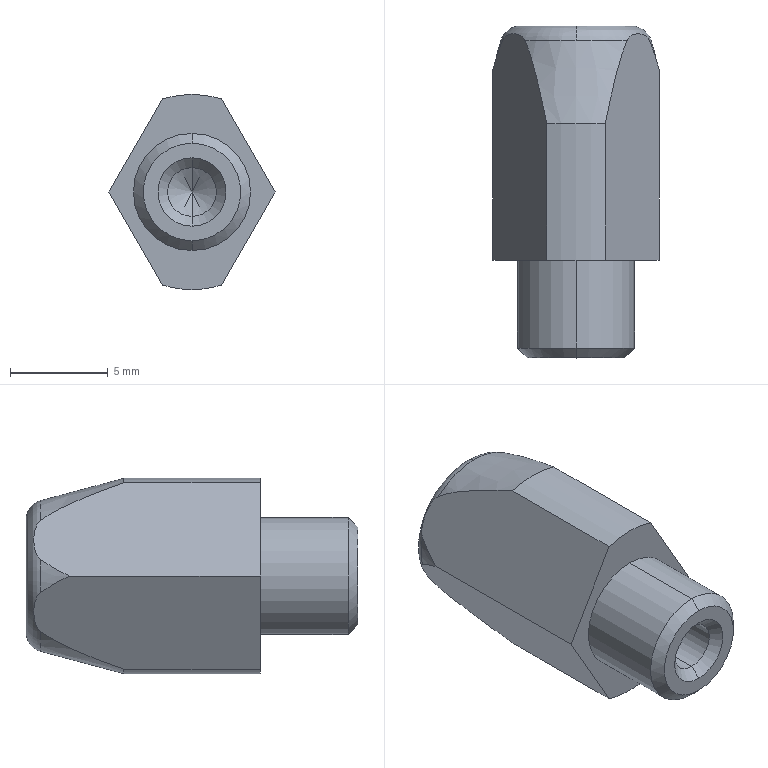Component | SolidWorks | MA060.03.03-05-2 | 1 solid | 27 faces | box 8.51 x 17 x 10 mm | volume 740 mm3 | cone 11 | cylinder 7 | plane 7 | torus 2 | commonest cylinder face diameters 10 x3 2.5 x2 6 x2 | material 45#
STEP:
#1=COLOUR_RGB('',0.7922,0.8196,0.9333);
#2=FILL_AREA_STYLE_COLOUR('',#1);
#3=FILL_AREA_STYLE('',(#2));
#4=SURFACE_STYLE_FILL_AREA(#3);
#5=SURFACE_SIDE_STYLE('',(#4));
#6=SURFACE_STYLE_USAGE(.BOTH.,#5);
#7=PRESENTATION_STYLE_ASSIGNMENT((#6));
#8=CARTESIAN_POINT('',(1.614,3.516,-0.1519));
#9=VERTEX_POINT('',#8);
#10=CARTESIAN_POINT('',(1.717,3.516,-0.1117));
#11=VERTEX_POINT('',#10);
#12=CARTESIAN_POINT('',(1.614,3.516,-0.));
#13=DIRECTION('',(0.,-1.,0.));
#14=DIRECTION('',(0.,0.,1.));
#15=AXIS2_PLACEMENT_3D('',#12,#13,#14);
#16=CIRCLE('',#15,0.1519);
#17=EDGE_CURVE('',#9,#11,#16,.T.);
#18=ORIENTED_EDGE('',*,*,#17,.F.);
#19=CARTESIAN_POINT('',(1.614,3.545,-0.1139));
#20=VERTEX_POINT('',#19);
#21=CARTESIAN_POINT('',(1.614,3.506,-0.1139));
#22=DIRECTION('',(1.,0.,0.));
#23=DIRECTION('',(0.,0.,-1.));
#24=AXIS2_PLACEMENT_3D('',#21,#22,#23);
#25=CIRCLE('',#24,0.03937);
#26=EDGE_CURVE('',#9,#20,#25,.T.);
#27=ORIENTED_EDGE('',*,*,#26,.T.);
#28=CARTESIAN_POINT('',(1.614,3.545,0.1139));
#29=VERTEX_POINT('',#28);
#30=CARTESIAN_POINT('',(1.614,3.545,-0.));
#31=DIRECTION('',(0.,1.,0.));
#32=DIRECTION('',(0.,0.,1.));
#33=AXIS2_PLACEMENT_3D('',#30,#31,#32);
#34=CIRCLE('',#33,0.1139);
#35=EDGE_CURVE('',#29,#20,#34,.T.);
#36=ORIENTED_EDGE('',*,*,#35,.F.);
#37=CARTESIAN_POINT('',(1.614,3.516,0.1519));
#38=VERTEX_POINT('',#37);
#39=CARTESIAN_POINT('',(1.614,3.506,0.1139));
#40=DIRECTION('',(-1.,0.,0.));
#41=DIRECTION('',(0.,0.,1.));
#42=AXIS2_PLACEMENT_3D('',#39,#40,#41);
#43=CIRCLE('',#42,0.03937);
#44=EDGE_CURVE('',#38,#29,#43,.T.);
#45=ORIENTED_EDGE('',*,*,#44,.F.);
#46=CARTESIAN_POINT('',(1.717,3.516,0.1117));
#47=VERTEX_POINT('',#46);
#48=CARTESIAN_POINT('',(1.614,3.516,-0.));
#49=DIRECTION('',(0.,-1.,0.));
#50=DIRECTION('',(0.,0.,1.));
#51=AXIS2_PLACEMENT_3D('',#48,#49,#50);
#52=CIRCLE('',#51,0.1519);
#53=EDGE_CURVE('',#47,#38,#52,.T.);
#54=ORIENTED_EDGE('',*,*,#53,.F.);
#55=CARTESIAN_POINT('',(1.762,3.516,0.03335));
#56=VERTEX_POINT('',#55);
#57=CARTESIAN_POINT('',(1.762,3.516,0.03335));
#58=CARTESIAN_POINT('',(1.761,3.519,0.03573));
#59=CARTESIAN_POINT('',(1.759,3.521,0.0387));
#60=CARTESIAN_POINT('',(1.756,3.525,0.04504));
#61=CARTESIAN_POINT('',(1.754,3.526,0.04835));
#62=CARTESIAN_POINT('',(1.748,3.529,0.05852));
#63=CARTESIAN_POINT('',(1.744,3.53,0.06554));
#64=CARTESIAN_POINT('',(1.736,3.53,0.07943));
#65=CARTESIAN_POINT('',(1.732,3.529,0.08647));
#66=CARTESIAN_POINT('',(1.726,3.526,0.09665));
#67=CARTESIAN_POINT('',(1.724,3.525,0.1));
#68=CARTESIAN_POINT('',(1.72,3.521,0.1063));
#69=CARTESIAN_POINT('',(1.719,3.519,0.1093));
#70=CARTESIAN_POINT('',(1.717,3.516,0.1117));
#71=B_SPLINE_CURVE_WITH_KNOTS('',3,(#57,#58,#59,#60,#61,#62,#63,#64,#65,#66,#67,#68,#69,#70),.UNSPECIFIED.,.F.,.F.,(4,2,2,2,2,2,4),(0.,0.0003075,0.0006151,0.00123,0.001845,0.002153,0.00246),.UNSPECIFIED.);
#72=EDGE_CURVE('',#56,#47,#71,.T.);
#73=ORIENTED_EDGE('',*,*,#72,.F.);
#74=CARTESIAN_POINT('',(1.762,3.516,-0.03335));
#75=VERTEX_POINT('',#74);
#76=CARTESIAN_POINT('',(1.614,3.516,-0.));
#77=DIRECTION('',(0.,-1.,0.));
#78=DIRECTION('',(0.,0.,1.));
#79=AXIS2_PLACEMENT_3D('',#76,#77,#78);
#80=CIRCLE('',#79,0.1519);
#81=EDGE_CURVE('',#75,#56,#80,.T.);
#82=ORIENTED_EDGE('',*,*,#81,.F.);
#83=CARTESIAN_POINT('',(1.717,3.516,-0.1117));
#84=CARTESIAN_POINT('',(1.719,3.519,-0.1093));
#85=CARTESIAN_POINT('',(1.72,3.521,-0.1063));
#86=CARTESIAN_POINT('',(1.724,3.525,-0.1));
#87=CARTESIAN_POINT('',(1.726,3.526,-0.09669));
#88=CARTESIAN_POINT('',(1.732,3.529,-0.08651));
#89=CARTESIAN_POINT('',(1.736,3.53,-0.07949));
#90=CARTESIAN_POINT('',(1.744,3.53,-0.06561));
#91=CARTESIAN_POINT('',(1.748,3.529,-0.05856));
#92=CARTESIAN_POINT('',(1.754,3.526,-0.04838));
#93=CARTESIAN_POINT('',(1.756,3.525,-0.04502));
#94=CARTESIAN_POINT('',(1.759,3.521,-0.03873));
#95=CARTESIAN_POINT('',(1.761,3.519,-0.03572));
#96=CARTESIAN_POINT('',(1.762,3.516,-0.03335));
#97=B_SPLINE_CURVE_WITH_KNOTS('',3,(#83,#84,#85,#86,#87,#88,#89,#90,#91,#92,#93,#94,#95,#96),.UNSPECIFIED.,.F.,.F.,(4,2,2,2,2,2,4),(0.,0.0003075,0.0006151,0.00123,0.001845,0.002153,0.00246),.UNSPECIFIED.);
#98=EDGE_CURVE('',#11,#75,#97,.T.);
#99=ORIENTED_EDGE('',*,*,#98,.F.);
#100=EDGE_LOOP('',(#18,#27,#36,#45,#54,#73,#82,#99));
#101=FACE_OUTER_BOUND('',#100,.T.);
#102=CARTESIAN_POINT('',(1.614,3.506,-0.));
#103=DIRECTION('',(0.,1.,0.));
#104=DIRECTION('',(0.,0.,1.));
#105=AXIS2_PLACEMENT_3D('',#102,#103,#104);
#106=TOROIDAL_SURFACE('',#105,0.1139,0.03937);
#107=ADVANCED_FACE('',(#101),#106,.T.);
#108=CARTESIAN_POINT('',(1.614,2.896,0.04921));
#109=VERTEX_POINT('',#108);
#110=CARTESIAN_POINT('',(1.614,2.896,-0.04921));
#111=VERTEX_POINT('',#110);
#112=CARTESIAN_POINT('',(1.614,2.896,-0.));
#113=DIRECTION('',(0.,-1.,0.));
#114=DIRECTION('',(0.,0.,-1.));
#115=AXIS2_PLACEMENT_3D('',#112,#113,#114);
#116=CIRCLE('',#115,0.04921);
#117=EDGE_CURVE('',#109,#111,#116,.T.);
#118=ORIENTED_EDGE('',*,*,#117,.F.);
#119=CARTESIAN_POINT('',(1.614,2.876,0.0689));
#120=VERTEX_POINT('',#119);
#121=CARTESIAN_POINT('',(1.614,2.896,0.04921));
#122=DIRECTION('',(0.,-0.7071,0.7071));
#123=VECTOR('',#122,39.37);
#124=LINE('',#121,#123);
#125=EDGE_CURVE('',#109,#120,#124,.T.);
#126=ORIENTED_EDGE('',*,*,#125,.T.);
#127=CARTESIAN_POINT('',(1.614,2.876,-0.0689));
#128=VERTEX_POINT('',#127);
#129=CARTESIAN_POINT('',(1.614,2.876,-0.));
#130=DIRECTION('',(0.,1.,0.));
#131=DIRECTION('',(0.,0.,-1.));
#132=AXIS2_PLACEMENT_3D('',#129,#130,#131);
#133=CIRCLE('',#132,0.0689);
#134=EDGE_CURVE('',#128,#120,#133,.T.);
#135=ORIENTED_EDGE('',*,*,#134,.F.);
#136=CARTESIAN_POINT('',(1.614,2.896,-0.04921));
#137=DIRECTION('',(0.,-0.7071,-0.7071));
#138=VECTOR('',#137,39.37);
#139=LINE('',#136,#138);
#140=EDGE_CURVE('',#111,#128,#139,.T.);
#141=ORIENTED_EDGE('',*,*,#140,.F.);
#142=EDGE_LOOP('',(#118,#126,#135,#141));
#143=FACE_OUTER_BOUND('',#142,.T.);
#144=CARTESIAN_POINT('',(1.614,2.896,-0.));
#145=DIRECTION('',(0.,-1.,0.));
#146=DIRECTION('',(0.,0.,-1.));
#147=AXIS2_PLACEMENT_3D('',#144,#145,#146);
#148=CONICAL_SURFACE('',#147,0.04921,0.7854);
#149=ADVANCED_FACE('',(#143),#148,.F.);
#150=CARTESIAN_POINT('',(1.614,2.876,-0.09843));
#151=VERTEX_POINT('',#150);
#152=CARTESIAN_POINT('',(1.614,2.876,0.09843));
#153=VERTEX_POINT('',#152);
#154=CARTESIAN_POINT('',(1.614,2.876,-0.));
#155=DIRECTION('',(0.,-1.,0.));
#156=DIRECTION('',(0.,0.,-1.));
#157=AXIS2_PLACEMENT_3D('',#154,#155,#156);
#158=CIRCLE('',#157,0.09843);
#159=EDGE_CURVE('',#151,#153,#158,.T.);
#160=ORIENTED_EDGE('',*,*,#159,.F.);
#161=CARTESIAN_POINT('',(1.614,2.896,-0.1181));
#162=VERTEX_POINT('',#161);
#163=CARTESIAN_POINT('',(1.614,2.876,-0.09843));
#164=DIRECTION('',(0.,0.7071,-0.7071));
#165=VECTOR('',#164,39.37);
#166=LINE('',#163,#165);
#167=EDGE_CURVE('',#151,#162,#166,.T.);
#168=ORIENTED_EDGE('',*,*,#167,.T.);
#169=CARTESIAN_POINT('',(1.614,2.896,0.1181));
#170=VERTEX_POINT('',#169);
#171=CARTESIAN_POINT('',(1.614,2.896,-0.));
#172=DIRECTION('',(0.,1.,0.));
#173=DIRECTION('',(0.,0.,-1.));
#174=AXIS2_PLACEMENT_3D('',#171,#172,#173);
#175=CIRCLE('',#174,0.1181);
#176=EDGE_CURVE('',#170,#162,#175,.T.);
#177=ORIENTED_EDGE('',*,*,#176,.F.);
#178=CARTESIAN_POINT('',(1.614,2.876,0.09843));
#179=DIRECTION('',(0.,0.7071,0.7071));
#180=VECTOR('',#179,39.37);
#181=LINE('',#178,#180);
#182=EDGE_CURVE('',#153,#170,#181,.T.);
#183=ORIENTED_EDGE('',*,*,#182,.F.);
#184=EDGE_LOOP('',(#160,#168,#177,#183));
#185=FACE_OUTER_BOUND('',#184,.T.);
#186=CARTESIAN_POINT('',(1.614,2.876,-0.));
#187=DIRECTION('',(0.,1.,0.));
#188=DIRECTION('',(0.,0.,1.));
#189=AXIS2_PLACEMENT_3D('',#186,#187,#188);
#190=CONICAL_SURFACE('',#189,0.09843,0.7854);
#191=ADVANCED_FACE('',(#185),#190,.T.);
#192=CARTESIAN_POINT('',(1.614,3.171,0.04921));
#193=VERTEX_POINT('',#192);
#194=CARTESIAN_POINT('',(1.614,3.171,-0.04921));
#195=VERTEX_POINT('',#194);
#196=CARTESIAN_POINT('',(1.614,3.171,-0.));
#197=DIRECTION('',(0.,-1.,0.));
#198=DIRECTION('',(0.,0.,-1.));
#199=AXIS2_PLACEMENT_3D('',#196,#197,#198);
#200=CIRCLE('',#199,0.04921);
#201=EDGE_CURVE('',#193,#195,#200,.T.);
#202=ORIENTED_EDGE('',*,*,#201,.F.);
#203=CARTESIAN_POINT('',(1.614,2.876,0.04921));
#204=DIRECTION('',(0.,-1.,0.));
#205=VECTOR('',#204,39.37);
#206=LINE('',#203,#205);
#207=EDGE_CURVE('',#193,#109,#206,.T.);
#208=ORIENTED_EDGE('',*,*,#207,.T.);
#209=ORIENTED_EDGE('',*,*,#117,.T.);
#210=CARTESIAN_POINT('',(1.614,2.876,-0.04921));
#211=DIRECTION('',(0.,-1.,0.));
#212=VECTOR('',#211,39.37);
#213=LINE('',#210,#212);
#214=EDGE_CURVE('',#195,#111,#213,.T.);
#215=ORIENTED_EDGE('',*,*,#214,.F.);
#216=EDGE_LOOP('',(#202,#208,#209,#215));
#217=FACE_OUTER_BOUND('',#216,.T.);
#218=CARTESIAN_POINT('',(1.614,2.876,-0.));
#219=DIRECTION('',(0.,-1.,0.));
#220=DIRECTION('',(0.,0.,-1.));
#221=AXIS2_PLACEMENT_3D('',#218,#219,#220);
#222=CYLINDRICAL_SURFACE('',#221,0.04921);
#223=ADVANCED_FACE('',(#217),#222,.F.);
#224=CARTESIAN_POINT('',(1.614,3.201,-0.));
#225=VERTEX_POINT('',#224);
#226=CARTESIAN_POINT('',(1.614,3.171,-0.04921));
#227=DIRECTION('',(0.,-0.515,-0.8572));
#228=VECTOR('',#227,39.37);
#229=LINE('',#226,#228);
#230=EDGE_CURVE('',#225,#195,#229,.T.);
#231=ORIENTED_EDGE('',*,*,#230,.F.);
#232=CARTESIAN_POINT('',(1.614,3.171,0.04921));
#233=DIRECTION('',(0.,-0.515,0.8572));
#234=VECTOR('',#233,39.37);
#235=LINE('',#232,#234);
#236=EDGE_CURVE('',#225,#193,#235,.T.);
#237=ORIENTED_EDGE('',*,*,#236,.T.);
#238=ORIENTED_EDGE('',*,*,#201,.T.);
#239=EDGE_LOOP('',(#231,#237,#238));
#240=FACE_OUTER_BOUND('',#239,.T.);
#241=CARTESIAN_POINT('',(1.614,3.171,-0.));
#242=DIRECTION('',(0.,-1.,0.));
#243=DIRECTION('',(0.,0.,-1.));
#244=AXIS2_PLACEMENT_3D('',#241,#242,#243);
#245=CONICAL_SURFACE('',#244,0.04921,1.03);
#246=ADVANCED_FACE('',(#240),#245,.F.);
#247=CARTESIAN_POINT('',(1.614,3.073,-0.1181));
#248=VERTEX_POINT('',#247);
#249=CARTESIAN_POINT('',(1.614,3.073,0.1181));
#250=VERTEX_POINT('',#249);
#251=CARTESIAN_POINT('',(1.614,3.073,-0.));
#252=DIRECTION('',(0.,-1.,0.));
#253=DIRECTION('',(0.,0.,-1.));
#254=AXIS2_PLACEMENT_3D('',#251,#252,#253);
#255=CIRCLE('',#254,0.1181);
#256=EDGE_CURVE('',#248,#250,#255,.T.);
#257=ORIENTED_EDGE('',*,*,#256,.T.);
#258=CARTESIAN_POINT('',(1.614,2.876,0.1181));
#259=DIRECTION('',(0.,-1.,0.));
#260=VECTOR('',#259,39.37);
#261=LINE('',#258,#260);
#262=EDGE_CURVE('',#250,#170,#261,.T.);
#263=ORIENTED_EDGE('',*,*,#262,.T.);
#264=ORIENTED_EDGE('',*,*,#176,.T.);
#265=CARTESIAN_POINT('',(1.614,2.876,-0.1181));
#266=DIRECTION('',(0.,-1.,0.));
#267=VECTOR('',#266,39.37);
#268=LINE('',#265,#267);
#269=EDGE_CURVE('',#248,#162,#268,.T.);
#270=ORIENTED_EDGE('',*,*,#269,.F.);
#271=EDGE_LOOP('',(#257,#263,#264,#270));
#272=FACE_OUTER_BOUND('',#271,.T.);
#273=CARTESIAN_POINT('',(1.614,2.876,-0.));
#274=DIRECTION('',(0.,-1.,0.));
#275=DIRECTION('',(0.,0.,-1.));
#276=AXIS2_PLACEMENT_3D('',#273,#274,#275);
#277=CYLINDRICAL_SURFACE('',#276,0.1181);
#278=ADVANCED_FACE('',(#272),#277,.T.);
#279=CARTESIAN_POINT('',(1.555,3.349,-0.1878));
#280=VERTEX_POINT('',#279);
#281=CARTESIAN_POINT('',(1.614,3.349,-0.1969));
#282=VERTEX_POINT('',#281);
#283=CARTESIAN_POINT('',(1.614,3.349,-0.));
#284=DIRECTION('',(0.,-1.,0.));
#285=DIRECTION('',(0.,0.,1.));
#286=AXIS2_PLACEMENT_3D('',#283,#284,#285);
#287=CIRCLE('',#286,0.1969);
#288=EDGE_CURVE('',#280,#282,#287,.T.);
#289=ORIENTED_EDGE('',*,*,#288,.T.);
#290=CARTESIAN_POINT('',(1.614,3.073,-0.1969));
#291=VERTEX_POINT('',#290);
#292=CARTESIAN_POINT('',(1.614,2.876,-0.1969));
#293=DIRECTION('',(0.,-1.,0.));
#294=VECTOR('',#293,39.37);
#295=LINE('',#292,#294);
#296=EDGE_CURVE('',#282,#291,#295,.T.);
#297=ORIENTED_EDGE('',*,*,#296,.T.);
#298=CARTESIAN_POINT('',(1.555,3.073,-0.1878));
#299=VERTEX_POINT('',#298);
#300=CARTESIAN_POINT('',(1.614,3.073,-0.));
#301=DIRECTION('',(0.,-1.,0.));
#302=DIRECTION('',(0.,0.,-1.));
#303=AXIS2_PLACEMENT_3D('',#300,#301,#302);
#304=CIRCLE('',#303,0.1969);
#305=EDGE_CURVE('',#299,#291,#304,.T.);
#306=ORIENTED_EDGE('',*,*,#305,.F.);
#307=CARTESIAN_POINT('',(1.555,3.545,-0.1878));
#308=DIRECTION('',(0.,-1.,0.));
#309=VECTOR('',#308,39.37);
#310=LINE('',#307,#309);
#311=EDGE_CURVE('',#280,#299,#310,.T.);
#312=ORIENTED_EDGE('',*,*,#311,.F.);
#313=EDGE_LOOP('',(#289,#297,#306,#312));
#314=FACE_OUTER_BOUND('',#313,.T.);
#315=CARTESIAN_POINT('',(1.614,2.876,-0.));
#316=DIRECTION('',(0.,-1.,0.));
#317=DIRECTION('',(0.,0.,-1.));
#318=AXIS2_PLACEMENT_3D('',#315,#316,#317);
#319=CYLINDRICAL_SURFACE('',#318,0.1969);
#320=ADVANCED_FACE('',(#314),#319,.T.);
#321=CARTESIAN_POINT('',(1.511,3.516,-0.1117));
#322=VERTEX_POINT('',#321);
#323=CARTESIAN_POINT('',(1.614,3.516,-0.));
#324=DIRECTION('',(0.,-1.,0.));
#325=DIRECTION('',(0.,0.,1.));
#326=AXIS2_PLACEMENT_3D('',#323,#324,#325);
#327=CIRCLE('',#326,0.1519);
#328=EDGE_CURVE('',#322,#9,#327,.T.);
#329=ORIENTED_EDGE('',*,*,#328,.T.);
#330=CARTESIAN_POINT('',(1.614,3.349,-0.1969));
#331=DIRECTION('',(0.,-0.9659,-0.2588));
#332=VECTOR('',#331,39.37);
#333=LINE('',#330,#332);
#334=EDGE_CURVE('',#9,#282,#333,.T.);
#335=ORIENTED_EDGE('',*,*,#334,.T.);
#336=ORIENTED_EDGE('',*,*,#288,.F.);
#337=CARTESIAN_POINT('',(1.511,3.516,-0.1117));
#338=CARTESIAN_POINT('',(1.514,3.51,-0.1163));
#339=CARTESIAN_POINT('',(1.516,3.504,-0.1205));
#340=CARTESIAN_POINT('',(1.521,3.491,-0.1284));
#341=CARTESIAN_POINT('',(1.523,3.484,-0.1321));
#342=CARTESIAN_POINT('',(1.529,3.464,-0.1426));
#343=CARTESIAN_POINT('',(1.533,3.45,-0.1489));
#344=CARTESIAN_POINT('',(1.543,3.407,-0.167));
#345=CARTESIAN_POINT('',(1.549,3.378,-0.1777));
#346=CARTESIAN_POINT('',(1.555,3.349,-0.1878));
#347=B_SPLINE_CURVE_WITH_KNOTS('',3,(#337,#338,#339,#340,#341,#342,#343,#344,#345,#346),.UNSPECIFIED.,.F.,.F.,(4,2,2,2,4),(0.004488,0.005096,0.005705,0.006922,0.009356),.UNSPECIFIED.);
#348=EDGE_CURVE('',#322,#280,#347,.T.);
#349=ORIENTED_EDGE('',*,*,#348,.F.);
#350=EDGE_LOOP('',(#329,#335,#336,#349));
#351=FACE_OUTER_BOUND('',#350,.T.);
#352=CARTESIAN_POINT('',(1.614,3.349,-0.));
#353=DIRECTION('',(0.,-1.,0.));
#354=DIRECTION('',(0.,0.,-1.));
#355=AXIS2_PLACEMENT_3D('',#352,#353,#354);
#356=CONICAL_SURFACE('',#355,0.1969,0.2618);
#357=ADVANCED_FACE('',(#351),#356,.T.);
#358=ORIENTED_EDGE('',*,*,#334,.F.);
#359=ORIENTED_EDGE('',*,*,#17,.T.);
#360=CARTESIAN_POINT('',(1.673,3.349,-0.1878));
#361=VERTEX_POINT('',#360);
#362=CARTESIAN_POINT('',(1.673,3.349,-0.1878));
#363=CARTESIAN_POINT('',(1.679,3.378,-0.1777));
#364=CARTESIAN_POINT('',(1.685,3.407,-0.167));
#365=CARTESIAN_POINT('',(1.696,3.45,-0.149));
#366=CARTESIAN_POINT('',(1.699,3.464,-0.1426));
#367=CARTESIAN_POINT('',(1.707,3.491,-0.1285));
#368=CARTESIAN_POINT('',(1.712,3.504,-0.1209));
#369=CARTESIAN_POINT('',(1.717,3.516,-0.1117));
#370=B_SPLINE_CURVE_WITH_KNOTS('',3,(#362,#363,#364,#365,#366,#367,#368,#369),.UNSPECIFIED.,.F.,.F.,(4,2,2,4),(0.00000021,0.002413,0.00362,0.004826),.UNSPECIFIED.);
#371=EDGE_CURVE('',#361,#11,#370,.T.);
#372=ORIENTED_EDGE('',*,*,#371,.F.);
#373=CARTESIAN_POINT('',(1.614,3.349,-0.));
#374=DIRECTION('',(0.,-1.,0.));
#375=DIRECTION('',(0.,0.,1.));
#376=AXIS2_PLACEMENT_3D('',#373,#374,#375);
#377=CIRCLE('',#376,0.1969);
#378=EDGE_CURVE('',#282,#361,#377,.T.);
#379=ORIENTED_EDGE('',*,*,#378,.F.);
#380=EDGE_LOOP('',(#358,#359,#372,#379));
#381=FACE_OUTER_BOUND('',#380,.T.);
#382=CARTESIAN_POINT('',(1.614,3.349,-0.));
#383=DIRECTION('',(0.,-1.,0.));
#384=DIRECTION('',(0.,0.,-1.));
#385=AXIS2_PLACEMENT_3D('',#382,#383,#384);
#386=CONICAL_SURFACE('',#385,0.1969,0.2618);
#387=ADVANCED_FACE('',(#381),#386,.T.);
#388=CARTESIAN_POINT('',(1.782,3.458,-0.));
#389=VERTEX_POINT('',#388);
#390=CARTESIAN_POINT('',(1.762,3.516,-0.03335));
#391=CARTESIAN_POINT('',(1.766,3.508,-0.02659));
#392=CARTESIAN_POINT('',(1.77,3.498,-0.02073));
#393=CARTESIAN_POINT('',(1.776,3.479,-0.009814));
#394=CARTESIAN_POINT('',(1.779,3.468,-0.004775));
#395=CARTESIAN_POINT('',(1.782,3.458,-0.));
#396=B_SPLINE_CURVE_WITH_KNOTS('',3,(#390,#391,#392,#393,#394,#395),.UNSPECIFIED.,.F.,.F.,(4,2,4),(0.007528,0.008416,0.009304),.UNSPECIFIED.);
#397=EDGE_CURVE('',#75,#389,#396,.T.);
#398=ORIENTED_EDGE('',*,*,#397,.F.);
#399=ORIENTED_EDGE('',*,*,#81,.T.);
#400=CARTESIAN_POINT('',(1.782,3.458,-0.));
#401=CARTESIAN_POINT('',(1.779,3.468,0.004764));
#402=CARTESIAN_POINT('',(1.776,3.479,0.009778));
#403=CARTESIAN_POINT('',(1.77,3.498,0.02069));
#404=CARTESIAN_POINT('',(1.766,3.508,0.02661));
#405=CARTESIAN_POINT('',(1.762,3.516,0.03335));
#406=B_SPLINE_CURVE_WITH_KNOTS('',3,(#400,#401,#402,#403,#404,#405),.UNSPECIFIED.,.F.,.F.,(4,2,4),(0.00000049,0.0008857,0.001771),.UNSPECIFIED.);
#407=EDGE_CURVE('',#389,#56,#406,.T.);
#408=ORIENTED_EDGE('',*,*,#407,.F.);
#409=EDGE_LOOP('',(#398,#399,#408));
#410=FACE_OUTER_BOUND('',#409,.T.);
#411=CARTESIAN_POINT('',(1.614,3.349,-0.));
#412=DIRECTION('',(0.,-1.,0.));
#413=DIRECTION('',(0.,0.,-1.));
#414=AXIS2_PLACEMENT_3D('',#411,#412,#413);
#415=CONICAL_SURFACE('',#414,0.1969,0.2618);
#416=ADVANCED_FACE('',(#410),#415,.T.);
#417=CARTESIAN_POINT('',(1.673,3.349,0.1878));
#418=VERTEX_POINT('',#417);
#419=CARTESIAN_POINT('',(1.717,3.516,0.1117));
#420=CARTESIAN_POINT('',(1.714,3.51,0.1163));
#421=CARTESIAN_POINT('',(1.712,3.504,0.1205));
#422=CARTESIAN_POINT('',(1.708,3.491,0.1284));
#423=CARTESIAN_POINT('',(1.705,3.484,0.1321));
#424=CARTESIAN_POINT('',(1.699,3.464,0.1426));
#425=CARTESIAN_POINT('',(1.696,3.45,0.1489));
#426=CARTESIAN_POINT('',(1.685,3.407,0.167));
#427=CARTESIAN_POINT('',(1.679,3.378,0.1777));
#428=CARTESIAN_POINT('',(1.673,3.349,0.1878));
#429=B_SPLINE_CURVE_WITH_KNOTS('',3,(#419,#420,#421,#422,#423,#424,#425,#426,#427,#428),.UNSPECIFIED.,.F.,.F.,(4,2,2,2,4),(0.004488,0.005096,0.005705,0.006922,0.009356),.UNSPECIFIED.);
#430=EDGE_CURVE('',#47,#418,#429,.T.);
#431=ORIENTED_EDGE('',*,*,#430,.F.);
#432=ORIENTED_EDGE('',*,*,#53,.T.);
#433=CARTESIAN_POINT('',(1.511,3.516,0.1117));
#434=VERTEX_POINT('',#433);
#435=CARTESIAN_POINT('',(1.614,3.516,-0.));
#436=DIRECTION('',(0.,-1.,0.));
#437=DIRECTION('',(0.,0.,1.));
#438=AXIS2_PLACEMENT_3D('',#435,#436,#437);
#439=CIRCLE('',#438,0.1519);
#440=EDGE_CURVE('',#38,#434,#439,.T.);
#441=ORIENTED_EDGE('',*,*,#440,.T.);
#442=CARTESIAN_POINT('',(1.555,3.349,0.1878));
#443=VERTEX_POINT('',#442);
#444=CARTESIAN_POINT('',(1.555,3.349,0.1878));
#445=CARTESIAN_POINT('',(1.549,3.378,0.1777));
#446=CARTESIAN_POINT('',(1.543,3.407,0.167));
#447=CARTESIAN_POINT('',(1.533,3.45,0.149));
#448=CARTESIAN_POINT('',(1.529,3.464,0.1426));
#449=CARTESIAN_POINT('',(1.521,3.491,0.1285));
#450=CARTESIAN_POINT('',(1.517,3.504,0.1209));
#451=CARTESIAN_POINT('',(1.511,3.516,0.1117));
#452=B_SPLINE_CURVE_WITH_KNOTS('',3,(#444,#445,#446,#447,#448,#449,#450,#451),.UNSPECIFIED.,.F.,.F.,(4,2,2,4),(0.00000021,0.002413,0.00362,0.004826),.UNSPECIFIED.);
#453=EDGE_CURVE('',#443,#434,#452,.T.);
#454=ORIENTED_EDGE('',*,*,#453,.F.);
#455=CARTESIAN_POINT('',(1.614,3.349,-0.));
#456=DIRECTION('',(0.,-1.,0.));
#457=DIRECTION('',(0.,0.,1.));
#458=AXIS2_PLACEMENT_3D('',#455,#456,#457);
#459=CIRCLE('',#458,0.1969);
#460=EDGE_CURVE('',#418,#443,#459,.T.);
#461=ORIENTED_EDGE('',*,*,#460,.F.);
#462=EDGE_LOOP('',(#431,#432,#441,#454,#461));
#463=FACE_OUTER_BOUND('',#462,.T.);
#464=CARTESIAN_POINT('',(1.614,3.349,-0.));
#465=DIRECTION('',(0.,-1.,0.));
#466=DIRECTION('',(0.,0.,-1.));
#467=AXIS2_PLACEMENT_3D('',#464,#465,#466);
#468=CONICAL_SURFACE('',#467,0.1969,0.2618);
#469=ADVANCED_FACE('',(#463),#468,.T.);
#470=ORIENTED_EDGE('',*,*,#296,.F.);
#471=ORIENTED_EDGE('',*,*,#378,.T.);
#472=CARTESIAN_POINT('',(1.673,3.073,-0.1878));
#473=VERTEX_POINT('',#472);
#474=CARTESIAN_POINT('',(1.673,3.545,-0.1878));
#475=DIRECTION('',(0.,-1.,0.));
#476=VECTOR('',#475,39.37);
#477=LINE('',#474,#476);
#478=EDGE_CURVE('',#361,#473,#477,.T.);
#479=ORIENTED_EDGE('',*,*,#478,.T.);
#480=CARTESIAN_POINT('',(1.614,3.073,-0.));
#481=DIRECTION('',(0.,-1.,0.));
#482=DIRECTION('',(0.,0.,-1.));
#483=AXIS2_PLACEMENT_3D('',#480,#481,#482);
#484=CIRCLE('',#483,0.1969);
#485=EDGE_CURVE('',#291,#473,#484,.T.);
#486=ORIENTED_EDGE('',*,*,#485,.F.);
#487=EDGE_LOOP('',(#470,#471,#479,#486));
#488=FACE_OUTER_BOUND('',#487,.T.);
#489=CARTESIAN_POINT('',(1.614,2.876,-0.));
#490=DIRECTION('',(0.,-1.,0.));
#491=DIRECTION('',(0.,0.,-1.));
#492=AXIS2_PLACEMENT_3D('',#489,#490,#491);
#493=CYLINDRICAL_SURFACE('',#492,0.1969);
#494=ADVANCED_FACE('',(#488),#493,.T.);
#495=CARTESIAN_POINT('',(1.614,2.876,-0.));
#496=DIRECTION('',(0.,-1.,0.));
#497=DIRECTION('',(0.,0.,-1.));
#498=AXIS2_PLACEMENT_3D('',#495,#496,#497);
#499=CIRCLE('',#498,0.09843);
#500=EDGE_CURVE('',#153,#151,#499,.T.);
#501=ORIENTED_EDGE('',*,*,#500,.T.);
#502=ORIENTED_EDGE('',*,*,#159,.T.);
#503=EDGE_LOOP('',(#501,#502));
#504=FACE_OUTER_BOUND('',#503,.T.);
#505=ORIENTED_EDGE('',*,*,#134,.T.);
#506=CARTESIAN_POINT('',(1.614,2.876,-0.));
#507=DIRECTION('',(0.,1.,0.));
#508=DIRECTION('',(0.,0.,-1.));
#509=AXIS2_PLACEMENT_3D('',#506,#507,#508);
#510=CIRCLE('',#509,0.0689);
#511=EDGE_CURVE('',#120,#128,#510,.T.);
#512=ORIENTED_EDGE('',*,*,#511,.T.);
#513=EDGE_LOOP('',(#505,#512));
#514=FACE_BOUND('',#513,.T.);
#515=CARTESIAN_POINT('',(1.732,2.876,-0.));
#516=DIRECTION('',(0.,-1.,0.));
#517=DIRECTION('',(0.,0.,-1.));
#518=AXIS2_PLACEMENT_3D('',#515,#516,#517);
#519=PLANE('',#518);
#520=ADVANCED_FACE('',(#504,#514),#519,.T.);
#521=ORIENTED_EDGE('',*,*,#35,.T.);
#522=CARTESIAN_POINT('',(1.614,3.545,-0.));
#523=DIRECTION('',(0.,1.,0.));
#524=DIRECTION('',(0.,0.,1.));
#525=AXIS2_PLACEMENT_3D('',#522,#523,#524);
#526=CIRCLE('',#525,0.1139);
#527=EDGE_CURVE('',#20,#29,#526,.T.);
#528=ORIENTED_EDGE('',*,*,#527,.T.);
#529=EDGE_LOOP('',(#521,#528));
#530=FACE_OUTER_BOUND('',#529,.T.);
#531=CARTESIAN_POINT('',(1.614,3.545,-0.));
#532=DIRECTION('',(0.,1.,0.));
#533=DIRECTION('',(0.,0.,1.));
#534=AXIS2_PLACEMENT_3D('',#531,#532,#533);
#535=PLANE('',#534);
#536=ADVANCED_FACE('',(#530),#535,.T.);
#537=CARTESIAN_POINT('',(1.673,3.073,0.1878));
#538=VERTEX_POINT('',#537);
#539=CARTESIAN_POINT('',(1.673,3.545,0.1878));
#540=DIRECTION('',(0.,-1.,0.));
#541=VECTOR('',#540,39.37);
#542=LINE('',#539,#541);
#543=EDGE_CURVE('',#418,#538,#542,.T.);
#544=ORIENTED_EDGE('',*,*,#543,.F.);
#545=ORIENTED_EDGE('',*,*,#460,.T.);
#546=CARTESIAN_POINT('',(1.555,3.073,0.1878));
#547=VERTEX_POINT('',#546);
#548=CARTESIAN_POINT('',(1.555,3.545,0.1878));
#549=DIRECTION('',(0.,-1.,0.));
#550=VECTOR('',#549,39.37);
#551=LINE('',#548,#550);
#552=EDGE_CURVE('',#443,#547,#551,.T.);
#553=ORIENTED_EDGE('',*,*,#552,.T.);
#554=CARTESIAN_POINT('',(1.614,3.073,-0.));
#555=DIRECTION('',(0.,-1.,0.));
#556=DIRECTION('',(0.,0.,-1.));
#557=AXIS2_PLACEMENT_3D('',#554,#555,#556);
#558=CIRCLE('',#557,0.1969);
#559=EDGE_CURVE('',#538,#547,#558,.T.);
#560=ORIENTED_EDGE('',*,*,#559,.F.);
#561=EDGE_LOOP('',(#544,#545,#553,#560));
#562=FACE_OUTER_BOUND('',#561,.T.);
#563=CARTESIAN_POINT('',(1.614,2.876,-0.));
#564=DIRECTION('',(0.,-1.,0.));
#565=DIRECTION('',(0.,0.,-1.));
#566=AXIS2_PLACEMENT_3D('',#563,#564,#565);
#567=CYLINDRICAL_SURFACE('',#566,0.1969);
#568=ADVANCED_FACE('',(#562),#567,.T.);
#569=CARTESIAN_POINT('',(1.782,3.073,-0.));
#570=VERTEX_POINT('',#569);
#571=CARTESIAN_POINT('',(1.782,3.073,-0.));
#572=DIRECTION('',(-0.5,0.,-0.866));
#573=VECTOR('',#572,39.37);
#574=LINE('',#571,#573);
#575=EDGE_CURVE('',#570,#473,#574,.T.);
#576=ORIENTED_EDGE('',*,*,#575,.F.);
#577=CARTESIAN_POINT('',(1.673,3.073,0.1878));
#578=DIRECTION('',(0.5,0.,-0.866));
#579=VECTOR('',#578,39.37);
#580=LINE('',#577,#579);
#581=EDGE_CURVE('',#538,#570,#580,.T.);
#582=ORIENTED_EDGE('',*,*,#581,.F.);
#583=ORIENTED_EDGE('',*,*,#559,.T.);
#584=CARTESIAN_POINT('',(1.447,3.073,-0.));
#585=VERTEX_POINT('',#584);
#586=CARTESIAN_POINT('',(1.555,3.073,0.1878));
#587=DIRECTION('',(0.5,0.,0.866));
#588=VECTOR('',#587,39.37);
#589=LINE('',#586,#588);
#590=EDGE_CURVE('',#585,#547,#589,.T.);
#591=ORIENTED_EDGE('',*,*,#590,.F.);
#592=CARTESIAN_POINT('',(1.447,3.073,-0.));
#593=DIRECTION('',(-0.5,0.,0.866));
#594=VECTOR('',#593,39.37);
#595=LINE('',#592,#594);
#596=EDGE_CURVE('',#299,#585,#595,.T.);
#597=ORIENTED_EDGE('',*,*,#596,.F.);
#598=ORIENTED_EDGE('',*,*,#305,.T.);
#599=ORIENTED_EDGE('',*,*,#485,.T.);
#600=EDGE_LOOP('',(#576,#582,#583,#591,#597,#598,#599));
#601=FACE_OUTER_BOUND('',#600,.T.);
#602=ORIENTED_EDGE('',*,*,#256,.F.);
#603=CARTESIAN_POINT('',(1.614,3.073,-0.));
#604=DIRECTION('',(0.,-1.,0.));
#605=DIRECTION('',(0.,0.,-1.));
#606=AXIS2_PLACEMENT_3D('',#603,#604,#605);
#607=CIRCLE('',#606,0.1181);
#608=EDGE_CURVE('',#250,#248,#607,.T.);
#609=ORIENTED_EDGE('',*,*,#608,.F.);
#610=EDGE_LOOP('',(#602,#609));
#611=FACE_BOUND('',#610,.T.);
#612=CARTESIAN_POINT('',(1.811,3.073,-0.));
#613=DIRECTION('',(0.,-1.,0.));
#614=DIRECTION('',(0.,0.,-1.));
#615=AXIS2_PLACEMENT_3D('',#612,#613,#614);
#616=PLANE('',#615);
#617=ADVANCED_FACE('',(#601,#611),#616,.T.);
#618=ORIENTED_EDGE('',*,*,#262,.F.);
#619=ORIENTED_EDGE('',*,*,#608,.T.);
#620=ORIENTED_EDGE('',*,*,#269,.T.);
#621=CARTESIAN_POINT('',(1.614,2.896,-0.));
#622=DIRECTION('',(0.,1.,0.));
#623=DIRECTION('',(0.,0.,-1.));
#624=AXIS2_PLACEMENT_3D('',#621,#622,#623);
#625=CIRCLE('',#624,0.1181);
#626=EDGE_CURVE('',#162,#170,#625,.T.);
#627=ORIENTED_EDGE('',*,*,#626,.T.);
#628=EDGE_LOOP('',(#618,#619,#620,#627));
#629=FACE_OUTER_BOUND('',#628,.T.);
#630=CARTESIAN_POINT('',(1.614,2.876,-0.));
#631=DIRECTION('',(0.,-1.,0.));
#632=DIRECTION('',(0.,0.,-1.));
#633=AXIS2_PLACEMENT_3D('',#630,#631,#632);
#634=CYLINDRICAL_SURFACE('',#633,0.1181);
#635=ADVANCED_FACE('',(#629),#634,.T.);
#636=CARTESIAN_POINT('',(1.466,3.516,0.03335));
#637=VERTEX_POINT('',#636);
#638=CARTESIAN_POINT('',(1.447,3.458,-0.));
#639=VERTEX_POINT('',#638);
#640=CARTESIAN_POINT('',(1.466,3.516,0.03335));
#641=CARTESIAN_POINT('',(1.462,3.508,0.02659));
#642=CARTESIAN_POINT('',(1.459,3.498,0.02073));
#643=CARTESIAN_POINT('',(1.452,3.479,0.009814));
#644=CARTESIAN_POINT('',(1.449,3.468,0.004775));
#645=CARTESIAN_POINT('',(1.447,3.458,-0.));
#646=B_SPLINE_CURVE_WITH_KNOTS('',3,(#640,#641,#642,#643,#644,#645),.UNSPECIFIED.,.F.,.F.,(4,2,4),(0.007528,0.008416,0.009304),.UNSPECIFIED.);
#647=EDGE_CURVE('',#637,#639,#646,.T.);
#648=ORIENTED_EDGE('',*,*,#647,.F.);
#649=CARTESIAN_POINT('',(1.466,3.516,-0.03335));
#650=VERTEX_POINT('',#649);
#651=CARTESIAN_POINT('',(1.614,3.516,-0.));
#652=DIRECTION('',(0.,-1.,0.));
#653=DIRECTION('',(0.,0.,1.));
#654=AXIS2_PLACEMENT_3D('',#651,#652,#653);
#655=CIRCLE('',#654,0.1519);
#656=EDGE_CURVE('',#637,#650,#655,.T.);
#657=ORIENTED_EDGE('',*,*,#656,.T.);
#658=CARTESIAN_POINT('',(1.447,3.458,-0.));
#659=CARTESIAN_POINT('',(1.449,3.468,-0.004764));
#660=CARTESIAN_POINT('',(1.452,3.479,-0.009778));
#661=CARTESIAN_POINT('',(1.459,3.498,-0.02069));
#662=CARTESIAN_POINT('',(1.462,3.508,-0.02661));
#663=CARTESIAN_POINT('',(1.466,3.516,-0.03335));
#664=B_SPLINE_CURVE_WITH_KNOTS('',3,(#658,#659,#660,#661,#662,#663),.UNSPECIFIED.,.F.,.F.,(4,2,4),(0.00000049,0.0008857,0.001771),.UNSPECIFIED.);
#665=EDGE_CURVE('',#639,#650,#664,.T.);
#666=ORIENTED_EDGE('',*,*,#665,.F.);
#667=EDGE_LOOP('',(#648,#657,#666));
#668=FACE_OUTER_BOUND('',#667,.T.);
#669=CARTESIAN_POINT('',(1.614,3.349,-0.));
#670=DIRECTION('',(0.,-1.,0.));
#671=DIRECTION('',(0.,0.,-1.));
#672=AXIS2_PLACEMENT_3D('',#669,#670,#671);
#673=CONICAL_SURFACE('',#672,0.1969,0.2618);
#674=ADVANCED_FACE('',(#668),#673,.T.);
#675=ORIENTED_EDGE('',*,*,#236,.F.);
#676=ORIENTED_EDGE('',*,*,#230,.T.);
#677=CARTESIAN_POINT('',(1.614,3.171,-0.));
#678=DIRECTION('',(0.,-1.,0.));
#679=DIRECTION('',(0.,0.,-1.));
#680=AXIS2_PLACEMENT_3D('',#677,#678,#679);
#681=CIRCLE('',#680,0.04921);
#682=EDGE_CURVE('',#195,#193,#681,.T.);
#683=ORIENTED_EDGE('',*,*,#682,.T.);
#684=EDGE_LOOP('',(#675,#676,#683));
#685=FACE_OUTER_BOUND('',#684,.T.);
#686=CARTESIAN_POINT('',(1.614,3.171,-0.));
#687=DIRECTION('',(0.,-1.,0.));
#688=DIRECTION('',(0.,0.,-1.));
#689=AXIS2_PLACEMENT_3D('',#686,#687,#688);
#690=CONICAL_SURFACE('',#689,0.04921,1.03);
#691=ADVANCED_FACE('',(#685),#690,.F.);
#692=ORIENTED_EDGE('',*,*,#207,.F.);
#693=ORIENTED_EDGE('',*,*,#682,.F.);
#694=ORIENTED_EDGE('',*,*,#214,.T.);
#695=CARTESIAN_POINT('',(1.614,2.896,-0.));
#696=DIRECTION('',(0.,-1.,0.));
#697=DIRECTION('',(0.,0.,-1.));
#698=AXIS2_PLACEMENT_3D('',#695,#696,#697);
#699=CIRCLE('',#698,0.04921);
#700=EDGE_CURVE('',#111,#109,#699,.T.);
#701=ORIENTED_EDGE('',*,*,#700,.T.);
#702=EDGE_LOOP('',(#692,#693,#694,#701));
#703=FACE_OUTER_BOUND('',#702,.T.);
#704=CARTESIAN_POINT('',(1.614,2.876,-0.));
#705=DIRECTION('',(0.,-1.,0.));
#706=DIRECTION('',(0.,0.,-1.));
#707=AXIS2_PLACEMENT_3D('',#704,#705,#706);
#708=CYLINDRICAL_SURFACE('',#707,0.04921);
#709=ADVANCED_FACE('',(#703),#708,.F.);
#710=ORIENTED_EDGE('',*,*,#167,.F.);
#711=ORIENTED_EDGE('',*,*,#500,.F.);
#712=ORIENTED_EDGE('',*,*,#182,.T.);
#713=ORIENTED_EDGE('',*,*,#626,.F.);
#714=EDGE_LOOP('',(#710,#711,#712,#713));
#715=FACE_OUTER_BOUND('',#714,.T.);
#716=CARTESIAN_POINT('',(1.614,2.876,-0.));
#717=DIRECTION('',(0.,1.,0.));
#718=DIRECTION('',(0.,0.,1.));
#719=AXIS2_PLACEMENT_3D('',#716,#717,#718);
#720=CONICAL_SURFACE('',#719,0.09843,0.7854);
#721=ADVANCED_FACE('',(#715),#720,.T.);
#722=ORIENTED_EDGE('',*,*,#125,.F.);
#723=ORIENTED_EDGE('',*,*,#700,.F.);
#724=ORIENTED_EDGE('',*,*,#140,.T.);
#725=ORIENTED_EDGE('',*,*,#511,.F.);
#726=EDGE_LOOP('',(#722,#723,#724,#725));
#727=FACE_OUTER_BOUND('',#726,.T.);
#728=CARTESIAN_POINT('',(1.614,2.896,-0.));
#729=DIRECTION('',(0.,-1.,0.));
#730=DIRECTION('',(0.,0.,-1.));
#731=AXIS2_PLACEMENT_3D('',#728,#729,#730);
#732=CONICAL_SURFACE('',#731,0.04921,0.7854);
#733=ADVANCED_FACE('',(#727),#732,.F.);
#734=ORIENTED_EDGE('',*,*,#453,.T.);
#735=CARTESIAN_POINT('',(1.511,3.516,0.1117));
#736=CARTESIAN_POINT('',(1.51,3.519,0.1093));
#737=CARTESIAN_POINT('',(1.508,3.521,0.1063));
#738=CARTESIAN_POINT('',(1.504,3.525,0.1));
#739=CARTESIAN_POINT('',(1.503,3.526,0.09669));
#740=CARTESIAN_POINT('',(1.497,3.529,0.08651));
#741=CARTESIAN_POINT('',(1.493,3.53,0.07949));
#742=CARTESIAN_POINT('',(1.485,3.53,0.06561));
#743=CARTESIAN_POINT('',(1.481,3.529,0.05856));
#744=CARTESIAN_POINT('',(1.475,3.526,0.04838));
#745=CARTESIAN_POINT('',(1.473,3.525,0.04502));
#746=CARTESIAN_POINT('',(1.469,3.521,0.03873));
#747=CARTESIAN_POINT('',(1.467,3.519,0.03572));
#748=CARTESIAN_POINT('',(1.466,3.516,0.03335));
#749=B_SPLINE_CURVE_WITH_KNOTS('',3,(#735,#736,#737,#738,#739,#740,#741,#742,#743,#744,#745,#746,#747,#748),.UNSPECIFIED.,.F.,.F.,(4,2,2,2,2,2,4),(0.,0.0003075,0.0006151,0.00123,0.001845,0.002153,0.00246),.UNSPECIFIED.);
#750=EDGE_CURVE('',#434,#637,#749,.T.);
#751=ORIENTED_EDGE('',*,*,#750,.T.);
#752=ORIENTED_EDGE('',*,*,#647,.T.);
#753=CARTESIAN_POINT('',(1.447,3.545,-0.));
#754=DIRECTION('',(0.,-1.,0.));
#755=VECTOR('',#754,39.37);
#756=LINE('',#753,#755);
#757=EDGE_CURVE('',#639,#585,#756,.T.);
#758=ORIENTED_EDGE('',*,*,#757,.T.);
#759=ORIENTED_EDGE('',*,*,#590,.T.);
#760=ORIENTED_EDGE('',*,*,#552,.F.);
#761=EDGE_LOOP('',(#734,#751,#752,#758,#759,#760));
#762=FACE_OUTER_BOUND('',#761,.T.);
#763=CARTESIAN_POINT('',(1.555,3.545,0.1878));
#764=DIRECTION('',(0.866,0.,-0.5));
#765=DIRECTION('',(-0.5,0.,-0.866));
#766=AXIS2_PLACEMENT_3D('',#763,#764,#765);
#767=PLANE('',#766);
#768=ADVANCED_FACE('',(#762),#767,.F.);
#769=ORIENTED_EDGE('',*,*,#665,.T.);
#770=CARTESIAN_POINT('',(1.466,3.516,-0.03335));
#771=CARTESIAN_POINT('',(1.467,3.519,-0.03573));
#772=CARTESIAN_POINT('',(1.469,3.521,-0.0387));
#773=CARTESIAN_POINT('',(1.473,3.525,-0.04504));
#774=CARTESIAN_POINT('',(1.475,3.526,-0.04835));
#775=CARTESIAN_POINT('',(1.48,3.529,-0.05852));
#776=CARTESIAN_POINT('',(1.485,3.53,-0.06554));
#777=CARTESIAN_POINT('',(1.493,3.53,-0.07943));
#778=CARTESIAN_POINT('',(1.497,3.529,-0.08647));
#779=CARTESIAN_POINT('',(1.503,3.526,-0.09665));
#780=CARTESIAN_POINT('',(1.504,3.525,-0.1));
#781=CARTESIAN_POINT('',(1.508,3.521,-0.1063));
#782=CARTESIAN_POINT('',(1.51,3.519,-0.1093));
#783=CARTESIAN_POINT('',(1.511,3.516,-0.1117));
#784=B_SPLINE_CURVE_WITH_KNOTS('',3,(#770,#771,#772,#773,#774,#775,#776,#777,#778,#779,#780,#781,#782,#783),.UNSPECIFIED.,.F.,.F.,(4,2,2,2,2,2,4),(0.,0.0003075,0.0006151,0.00123,0.001845,0.002153,0.00246),.UNSPECIFIED.);
#785=EDGE_CURVE('',#650,#322,#784,.T.);
#786=ORIENTED_EDGE('',*,*,#785,.T.);
#787=ORIENTED_EDGE('',*,*,#348,.T.);
#788=ORIENTED_EDGE('',*,*,#311,.T.);
#789=ORIENTED_EDGE('',*,*,#596,.T.);
#790=ORIENTED_EDGE('',*,*,#757,.F.);
#791=EDGE_LOOP('',(#769,#786,#787,#788,#789,#790));
#792=FACE_OUTER_BOUND('',#791,.T.);
#793=CARTESIAN_POINT('',(1.447,3.545,-0.));
#794=DIRECTION('',(0.866,0.,0.5));
#795=DIRECTION('',(0.5,0.,-0.866));
#796=AXIS2_PLACEMENT_3D('',#793,#794,#795);
#797=PLANE('',#796);
#798=ADVANCED_FACE('',(#792),#797,.F.);
#799=ORIENTED_EDGE('',*,*,#371,.T.);
#800=ORIENTED_EDGE('',*,*,#98,.T.);
#801=ORIENTED_EDGE('',*,*,#397,.T.);
#802=CARTESIAN_POINT('',(1.782,3.545,-0.));
#803=DIRECTION('',(0.,-1.,0.));
#804=VECTOR('',#803,39.37);
#805=LINE('',#802,#804);
#806=EDGE_CURVE('',#389,#570,#805,.T.);
#807=ORIENTED_EDGE('',*,*,#806,.T.);
#808=ORIENTED_EDGE('',*,*,#575,.T.);
#809=ORIENTED_EDGE('',*,*,#478,.F.);
#810=EDGE_LOOP('',(#799,#800,#801,#807,#808,#809));
#811=FACE_OUTER_BOUND('',#810,.T.);
#812=CARTESIAN_POINT('',(1.782,3.545,-0.));
#813=DIRECTION('',(-0.866,0.,0.5));
#814=DIRECTION('',(0.5,0.,0.866));
#815=AXIS2_PLACEMENT_3D('',#812,#813,#814);
#816=PLANE('',#815);
#817=ADVANCED_FACE('',(#811),#816,.F.);
#818=ORIENTED_EDGE('',*,*,#407,.T.);
#819=ORIENTED_EDGE('',*,*,#72,.T.);
#820=ORIENTED_EDGE('',*,*,#430,.T.);
#821=ORIENTED_EDGE('',*,*,#543,.T.);
#822=ORIENTED_EDGE('',*,*,#581,.T.);
#823=ORIENTED_EDGE('',*,*,#806,.F.);
#824=EDGE_LOOP('',(#818,#819,#820,#821,#822,#823));
#825=FACE_OUTER_BOUND('',#824,.T.);
#826=CARTESIAN_POINT('',(1.673,3.545,0.1878));
#827=DIRECTION('',(-0.866,0.,-0.5));
#828=DIRECTION('',(-0.5,0.,0.866));
#829=AXIS2_PLACEMENT_3D('',#826,#827,#828);
#830=PLANE('',#829);
#831=ADVANCED_FACE('',(#825),#830,.F.);
#832=ORIENTED_EDGE('',*,*,#26,.F.);
#833=ORIENTED_EDGE('',*,*,#328,.F.);
#834=ORIENTED_EDGE('',*,*,#785,.F.);
#835=ORIENTED_EDGE('',*,*,#656,.F.);
#836=ORIENTED_EDGE('',*,*,#750,.F.);
#837=ORIENTED_EDGE('',*,*,#440,.F.);
#838=ORIENTED_EDGE('',*,*,#44,.T.);
#839=ORIENTED_EDGE('',*,*,#527,.F.);
#840=EDGE_LOOP('',(#832,#833,#834,#835,#836,#837,#838,#839));
#841=FACE_OUTER_BOUND('',#840,.T.);
#842=CARTESIAN_POINT('',(1.614,3.506,-0.));
#843=DIRECTION('',(0.,1.,0.));
#844=DIRECTION('',(0.,0.,1.));
#845=AXIS2_PLACEMENT_3D('',#842,#843,#844);
#846=TOROIDAL_SURFACE('',#845,0.1139,0.03937);
#847=ADVANCED_FACE('',(#841),#846,.T.);
#848=CLOSED_SHELL('',(#107,#149,#191,#223,#246,#278,#320,#357,#387,#416,#469,#494,#520,#536,#568,#617,#635,#674,#691,#709,#721,#733,#768,#798,#817,#831,#847));
#849=MANIFOLD_SOLID_BREP('',#848);
#850=STYLED_ITEM('',(#7),#849);
#851=(LENGTH_UNIT()NAMED_UNIT(*)SI_UNIT($,.METRE.));
#852=LENGTH_MEASURE_WITH_UNIT(LENGTH_MEASURE(0.0254),#851);
#853=DIMENSIONAL_EXPONENTS(1.,0.,0.,0.,0.,0.,0.);
#854=(CONVERSION_BASED_UNIT('',#852)LENGTH_UNIT()NAMED_UNIT(#853));
#855=UNCERTAINTY_MEASURE_WITH_UNIT(LENGTH_MEASURE(0.00001),#854,'','');
#856=(NAMED_UNIT(*)PLANE_ANGLE_UNIT()SI_UNIT($,.RADIAN.));
#857=(NAMED_UNIT(*)SI_UNIT($,.STERADIAN.)SOLID_ANGLE_UNIT());
#858=(GEOMETRIC_REPRESENTATION_CONTEXT(3)GLOBAL_UNCERTAINTY_ASSIGNED_CONTEXT((#855))GLOBAL_UNIT_ASSIGNED_CONTEXT((#854,#856,#857))REPRESENTATION_CONTEXT('',''));
#859=MECHANICAL_DESIGN_GEOMETRIC_PRESENTATION_REPRESENTATION('',(#850),#858);
#860=CARTESIAN_POINT('',(0.,0.,0.));
#861=DIRECTION('',(0.,0.,1.));
#862=DIRECTION('',(1.,0.,0.));
#863=AXIS2_PLACEMENT_3D('',#860,#861,#862);
#864=(LENGTH_UNIT()NAMED_UNIT(*)SI_UNIT($,.METRE.));
#865=LENGTH_MEASURE_WITH_UNIT(LENGTH_MEASURE(0.0254),#864);
#866=DIMENSIONAL_EXPONENTS(1.,0.,0.,0.,0.,0.,0.);
#867=(CONVERSION_BASED_UNIT('',#865)LENGTH_UNIT()NAMED_UNIT(#866));
#868=UNCERTAINTY_MEASURE_WITH_UNIT(LENGTH_MEASURE(0.00001),#867,'','');
#869=(NAMED_UNIT(*)PLANE_ANGLE_UNIT()SI_UNIT($,.RADIAN.));
#870=(NAMED_UNIT(*)SI_UNIT($,.STERADIAN.)SOLID_ANGLE_UNIT());
#871=(GEOMETRIC_REPRESENTATION_CONTEXT(3)GLOBAL_UNCERTAINTY_ASSIGNED_CONTEXT((#868))GLOBAL_UNIT_ASSIGNED_CONTEXT((#867,#869,#870))REPRESENTATION_CONTEXT('',''));
#872=ADVANCED_BREP_SHAPE_REPRESENTATION('',(#849,#863),#871);
#873=PRESENTATION_LAYER_ASSIGNMENT('','',(#850));